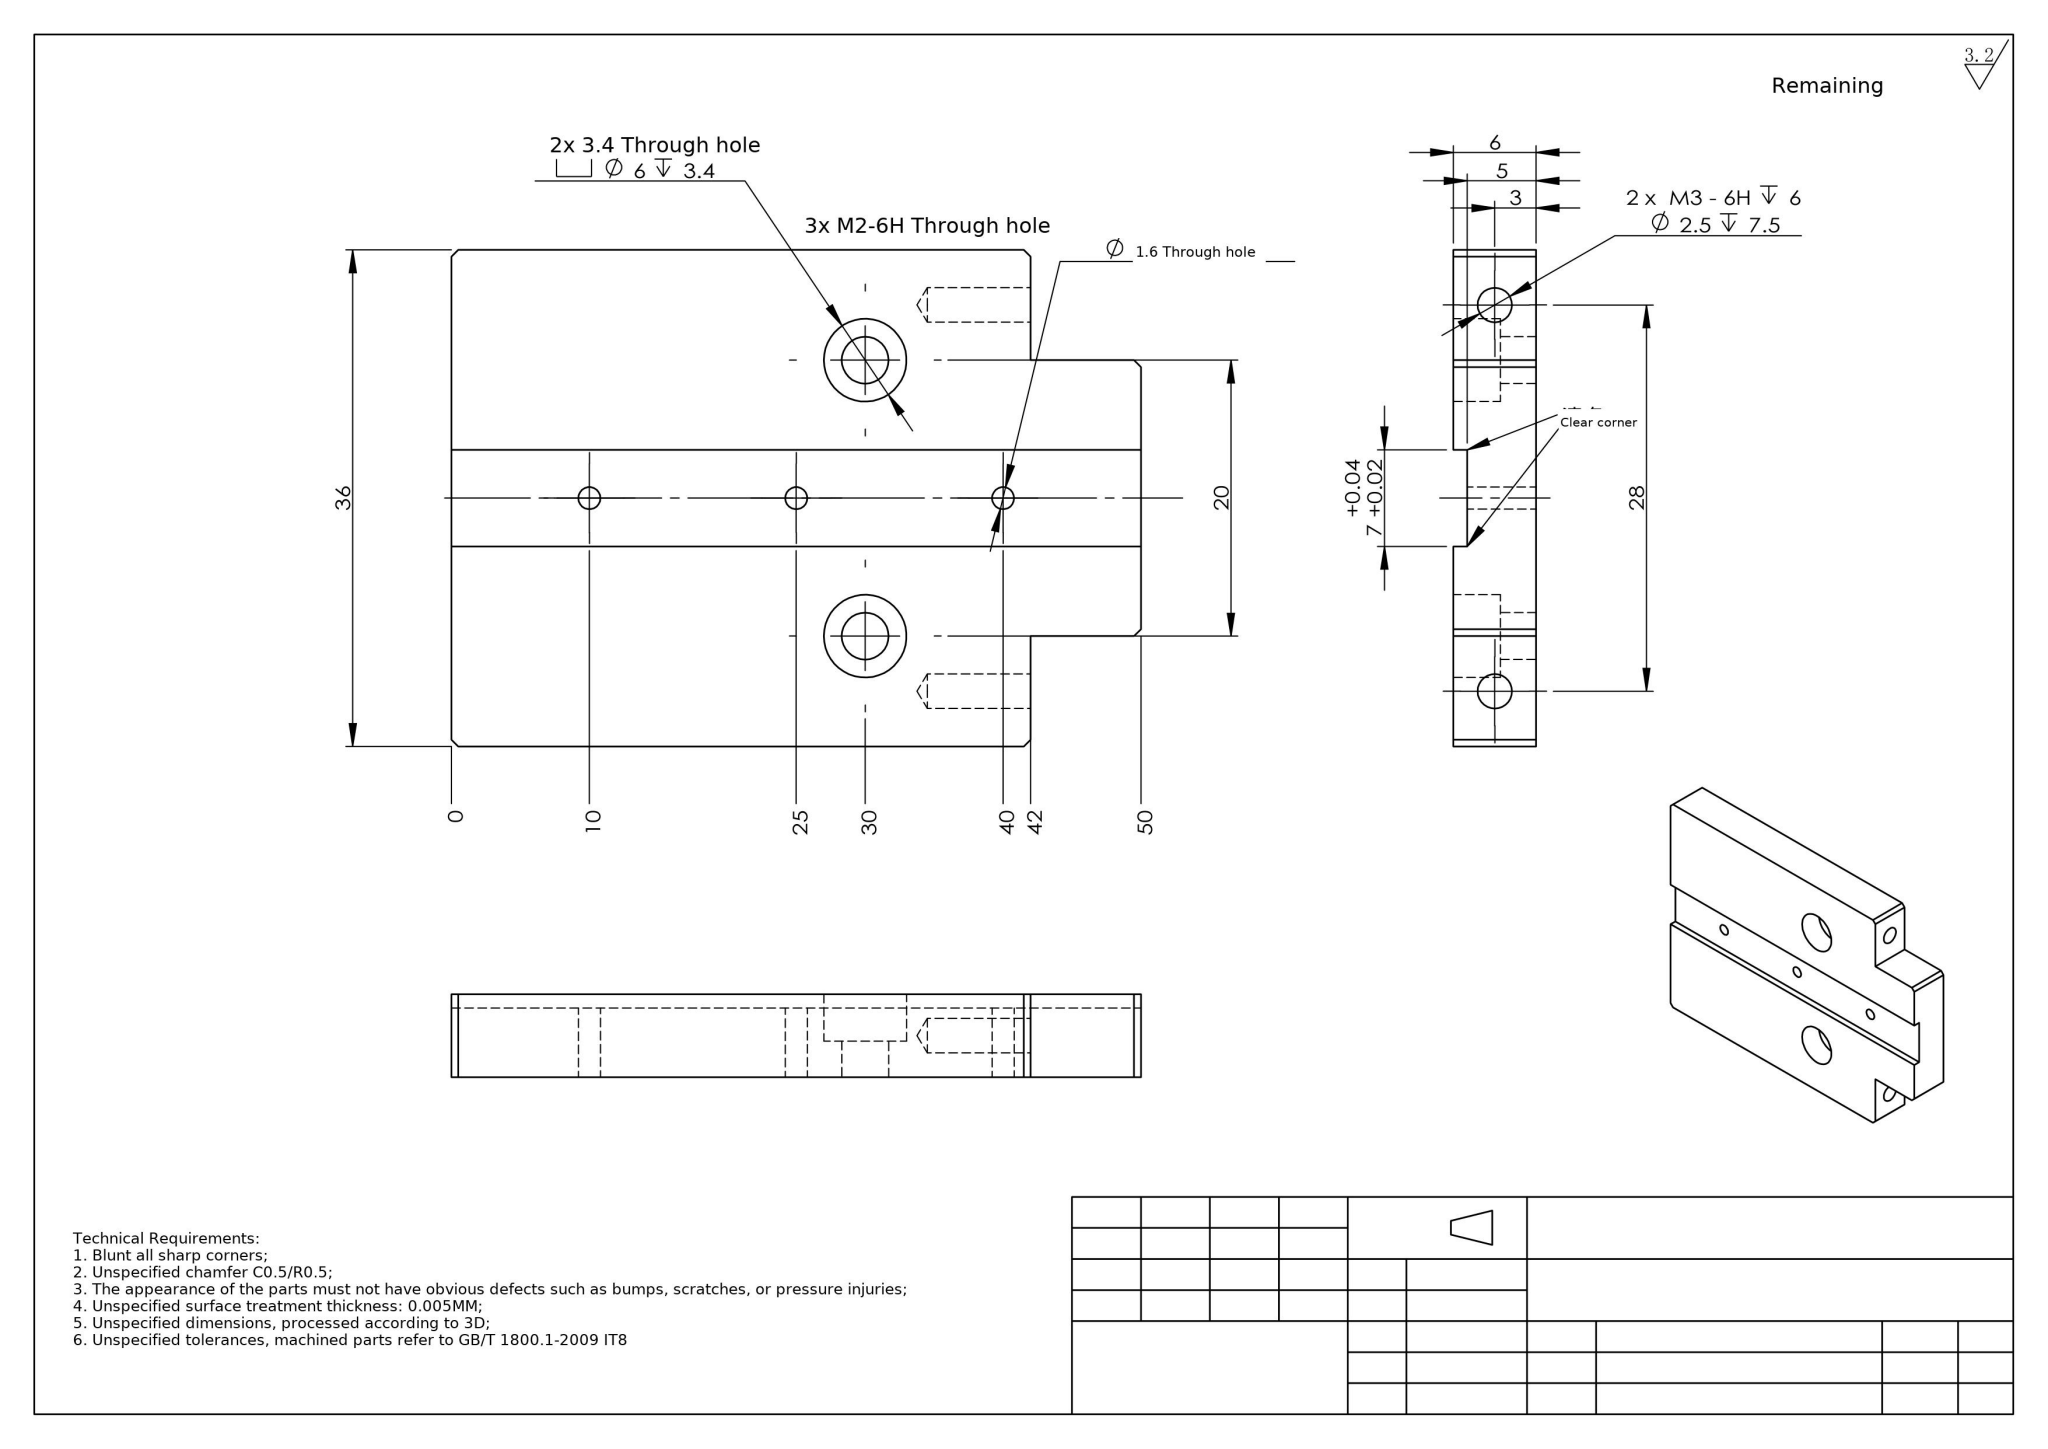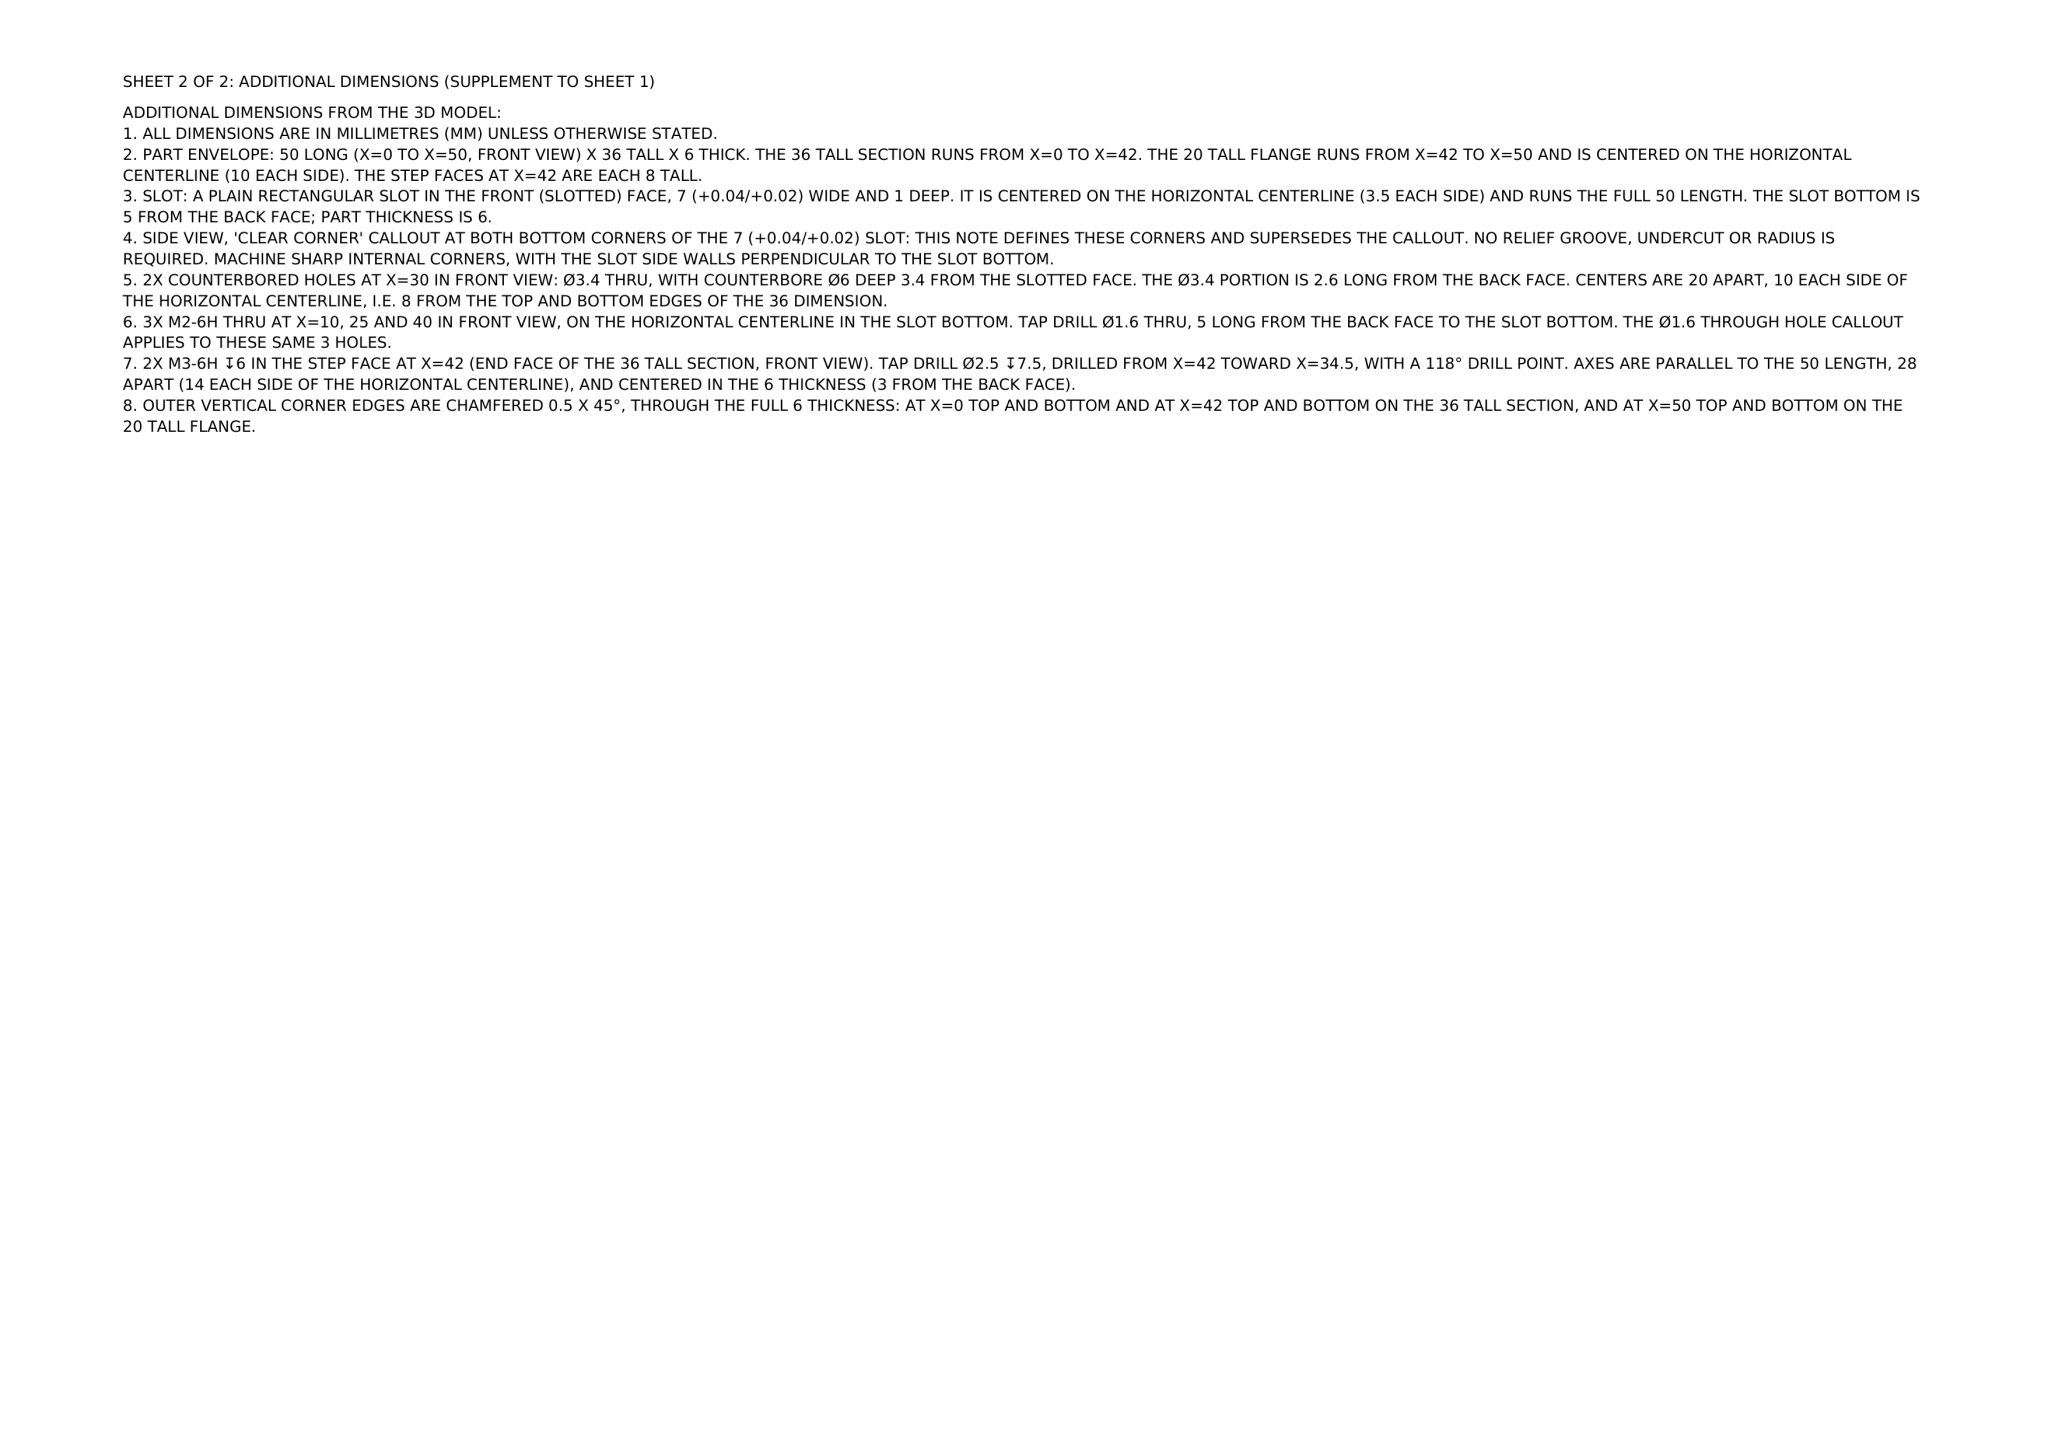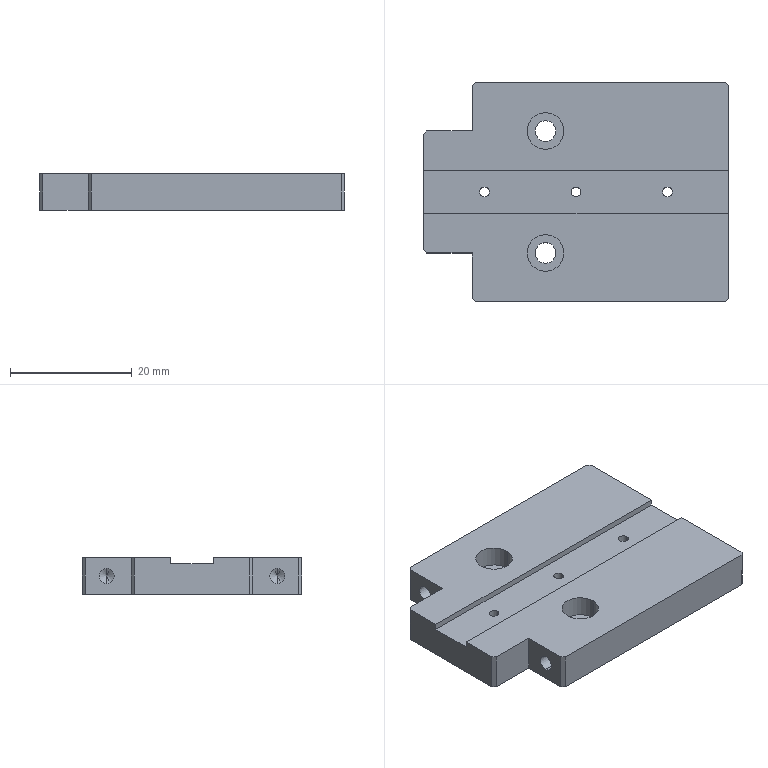Part | NX | mm | 1 solid | 44 faces | box 50 x 36 x 6 mm | volume 9332 mm3 | plane 22 | cylinder 18 | cone 4 | commonest cylinder face diameters 1.6 x6 2.5 x4 6 x4 3.4 x4